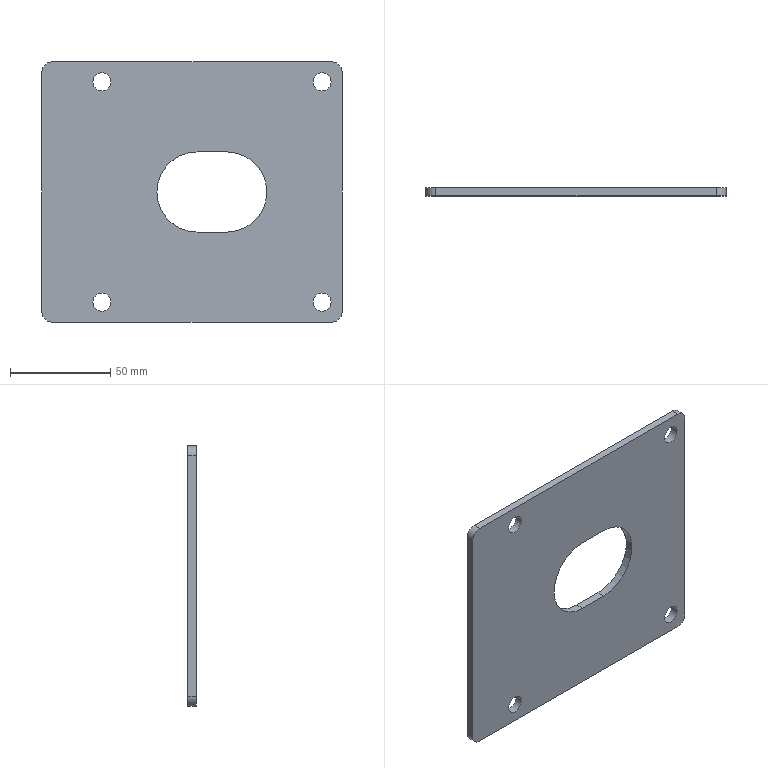Component | SolidWorks | CoverPlate.1_2-1 | 1 solid | 23 faces | box 150 x 4 x 130 mm | volume 69470 mm3 | cylinder 15 | plane 8 | commonest cylinder face diameters 9 x8 10 x4 40 x3
build123d program:
from build123d import *

# Parameters (mm, degrees)
SKETCH1_W           = 130
SKETCH1_H           = 150
BOSS_EXTRUDE1_DEPTH = 4
SKETCH2_R           = 4.5
CUT_EXTRUDE1_DEPTH  = 5
CUT_EXTRUDE2_DEPTH  = 5
FILLET1_R           = 5


with BuildPart() as part:
    # Sketch1 → Boss-Extrude1 (new body)
    with BuildSketch(Plane(origin=(0, 0, 0), x_dir=(1, 0, 0), z_dir=(0, 1, 0))):
        Rectangle(SKETCH1_W, SKETCH1_H)
    extrude(amount=BOSS_EXTRUDE1_DEPTH)

    # Sketch2 → Cut-Extrude1 (cut)
    with BuildSketch(Plane(origin=(0, 4, 0), x_dir=(1, 0, 0), z_dir=(0, 1, 0))):
        with Locations(Location((-55, 65, 0), (0, 0, 270))):
            Circle(SKETCH2_R)
        with Locations(Location((55, 65, 0), (0, 0, 270))):
            Circle(SKETCH2_R)
        with Locations(Location((55, -45, 0), (0, 0, 270))):
            Circle(SKETCH2_R)
        with Locations(Location((-55, -45, 0), (0, 0, 270))):
            Circle(SKETCH2_R)
    extrude(amount=-CUT_EXTRUDE1_DEPTH, mode=Mode.SUBTRACT)

    # Sketch3 → Cut-Extrude2 (cut)
    with BuildSketch(Plane(origin=(0, 4, 0), x_dir=(1, 0, 0), z_dir=(0, 1, 0))):
        with BuildLine():
            Line((-20, 2.5), (-20, 17.5))
            ThreePointArc((-20, 17.5), (0, 37.5), (20, 17.5))
            Line((20, 17.5), (20, 2.5))
            ThreePointArc((20, 2.5), (0, -17.5), (-20, 2.5))
        make_face()
    extrude(amount=-CUT_EXTRUDE2_DEPTH, mode=Mode.SUBTRACT)

    # Fillet1
    fillet1_edges = [part.edges().sort_by_distance(p)[0] for p in [
        (65, 2, 75),
        (-65, 2, 75),
        (-65, 2, -75),
        (65, 2, -75),
    ]]
    fillet(fillet1_edges, radius=FILLET1_R)


solid = part.part

# Placed as in the assembly
solid = solid.moved(Location((-10, 0, -0.4), (0, -90, 0)))
STEP:
#1=CARTESIAN_POINT('',(-1.083,-0.,-0.01575));
#2=VERTEX_POINT('',#1);
#3=CARTESIAN_POINT('',(-0.2953,-0.,0.7717));
#4=VERTEX_POINT('',#3);
#5=CARTESIAN_POINT('',(-0.2953,-0.,-0.01575));
#6=DIRECTION('',(0.,1.,-0.));
#7=DIRECTION('',(-1.,0.,-0.));
#8=AXIS2_PLACEMENT_3D('',#5,#6,#7);
#9=CIRCLE('',#8,0.7874);
#10=EDGE_CURVE('',#2,#4,#9,.T.);
#11=ORIENTED_EDGE('',*,*,#10,.F.);
#12=CARTESIAN_POINT('',(-1.083,0.1575,-0.01575));
#13=VERTEX_POINT('',#12);
#14=CARTESIAN_POINT('',(-1.083,-0.03937,-0.01575));
#15=DIRECTION('',(0.,1.,-0.));
#16=VECTOR('',#15,39.37);
#17=LINE('',#14,#16);
#18=EDGE_CURVE('',#2,#13,#17,.T.);
#19=ORIENTED_EDGE('',*,*,#18,.T.);
#20=CARTESIAN_POINT('',(-0.2953,0.1575,0.7717));
#21=VERTEX_POINT('',#20);
#22=CARTESIAN_POINT('',(-0.2953,0.1575,-0.01575));
#23=DIRECTION('',(0.,1.,-0.));
#24=DIRECTION('',(-1.,0.,-0.));
#25=AXIS2_PLACEMENT_3D('',#22,#23,#24);
#26=CIRCLE('',#25,0.7874);
#27=EDGE_CURVE('',#13,#21,#26,.T.);
#28=ORIENTED_EDGE('',*,*,#27,.T.);
#29=CARTESIAN_POINT('',(-0.2953,-0.03937,0.7717));
#30=DIRECTION('',(0.,1.,-0.));
#31=VECTOR('',#30,39.37);
#32=LINE('',#29,#31);
#33=EDGE_CURVE('',#4,#21,#32,.T.);
#34=ORIENTED_EDGE('',*,*,#33,.F.);
#35=EDGE_LOOP('',(#11,#19,#28,#34));
#36=FACE_OUTER_BOUND('',#35,.T.);
#37=CARTESIAN_POINT('',(-0.2953,-0.03937,-0.01575));
#38=DIRECTION('',(0.,1.,-0.));
#39=DIRECTION('',(-1.,0.,-0.));
#40=AXIS2_PLACEMENT_3D('',#37,#38,#39);
#41=CYLINDRICAL_SURFACE('',#40,0.7874);
#42=ADVANCED_FACE('',(#36),#41,.F.);
#43=CARTESIAN_POINT('',(-1.988,-0.,-2.181));
#44=VERTEX_POINT('',#43);
#45=CARTESIAN_POINT('',(-2.343,-0.,-2.181));
#46=VERTEX_POINT('',#45);
#47=CARTESIAN_POINT('',(-2.165,-0.,-2.181));
#48=DIRECTION('',(0.,1.,-0.));
#49=DIRECTION('',(-1.,0.,0.));
#50=AXIS2_PLACEMENT_3D('',#47,#48,#49);
#51=CIRCLE('',#50,0.1772);
#52=EDGE_CURVE('',#44,#46,#51,.T.);
#53=ORIENTED_EDGE('',*,*,#52,.F.);
#54=CARTESIAN_POINT('',(-1.988,0.1575,-2.181));
#55=VERTEX_POINT('',#54);
#56=CARTESIAN_POINT('',(-1.988,-0.03937,-2.181));
#57=DIRECTION('',(0.,1.,-0.));
#58=VECTOR('',#57,39.37);
#59=LINE('',#56,#58);
#60=EDGE_CURVE('',#44,#55,#59,.T.);
#61=ORIENTED_EDGE('',*,*,#60,.T.);
#62=CARTESIAN_POINT('',(-2.343,0.1575,-2.181));
#63=VERTEX_POINT('',#62);
#64=CARTESIAN_POINT('',(-2.165,0.1575,-2.181));
#65=DIRECTION('',(0.,1.,-0.));
#66=DIRECTION('',(1.,0.,0.));
#67=AXIS2_PLACEMENT_3D('',#64,#65,#66);
#68=CIRCLE('',#67,0.1772);
#69=EDGE_CURVE('',#55,#63,#68,.T.);
#70=ORIENTED_EDGE('',*,*,#69,.T.);
#71=CARTESIAN_POINT('',(-2.343,-0.03937,-2.181));
#72=DIRECTION('',(0.,1.,-0.));
#73=VECTOR('',#72,39.37);
#74=LINE('',#71,#73);
#75=EDGE_CURVE('',#46,#63,#74,.T.);
#76=ORIENTED_EDGE('',*,*,#75,.F.);
#77=EDGE_LOOP('',(#53,#61,#70,#76));
#78=FACE_OUTER_BOUND('',#77,.T.);
#79=CARTESIAN_POINT('',(-2.165,-0.03937,-2.181));
#80=DIRECTION('',(0.,1.,-0.));
#81=DIRECTION('',(-1.,0.,0.));
#82=AXIS2_PLACEMENT_3D('',#79,#80,#81);
#83=CYLINDRICAL_SURFACE('',#82,0.1772);
#84=ADVANCED_FACE('',(#78),#83,.F.);
#85=CARTESIAN_POINT('',(-1.988,-0.,2.15));
#86=VERTEX_POINT('',#85);
#87=CARTESIAN_POINT('',(-2.343,-0.,2.15));
#88=VERTEX_POINT('',#87);
#89=CARTESIAN_POINT('',(-2.165,-0.,2.15));
#90=DIRECTION('',(0.,1.,-0.));
#91=DIRECTION('',(-1.,0.,0.));
#92=AXIS2_PLACEMENT_3D('',#89,#90,#91);
#93=CIRCLE('',#92,0.1772);
#94=EDGE_CURVE('',#86,#88,#93,.T.);
#95=ORIENTED_EDGE('',*,*,#94,.F.);
#96=CARTESIAN_POINT('',(-1.988,0.1575,2.15));
#97=VERTEX_POINT('',#96);
#98=CARTESIAN_POINT('',(-1.988,-0.03937,2.15));
#99=DIRECTION('',(0.,1.,-0.));
#100=VECTOR('',#99,39.37);
#101=LINE('',#98,#100);
#102=EDGE_CURVE('',#86,#97,#101,.T.);
#103=ORIENTED_EDGE('',*,*,#102,.T.);
#104=CARTESIAN_POINT('',(-2.343,0.1575,2.15));
#105=VERTEX_POINT('',#104);
#106=CARTESIAN_POINT('',(-2.165,0.1575,2.15));
#107=DIRECTION('',(0.,1.,-0.));
#108=DIRECTION('',(-1.,0.,0.));
#109=AXIS2_PLACEMENT_3D('',#106,#107,#108);
#110=CIRCLE('',#109,0.1772);
#111=EDGE_CURVE('',#97,#105,#110,.T.);
#112=ORIENTED_EDGE('',*,*,#111,.T.);
#113=CARTESIAN_POINT('',(-2.343,-0.03937,2.15));
#114=DIRECTION('',(0.,1.,-0.));
#115=VECTOR('',#114,39.37);
#116=LINE('',#113,#115);
#117=EDGE_CURVE('',#88,#105,#116,.T.);
#118=ORIENTED_EDGE('',*,*,#117,.F.);
#119=EDGE_LOOP('',(#95,#103,#112,#118));
#120=FACE_OUTER_BOUND('',#119,.T.);
#121=CARTESIAN_POINT('',(-2.165,-0.03937,2.15));
#122=DIRECTION('',(0.,1.,-0.));
#123=DIRECTION('',(-1.,0.,0.));
#124=AXIS2_PLACEMENT_3D('',#121,#122,#123);
#125=CYLINDRICAL_SURFACE('',#124,0.1772);
#126=ADVANCED_FACE('',(#120),#125,.F.);
#127=CARTESIAN_POINT('',(2.343,-0.,2.15));
#128=VERTEX_POINT('',#127);
#129=CARTESIAN_POINT('',(1.988,-0.,2.15));
#130=VERTEX_POINT('',#129);
#131=CARTESIAN_POINT('',(2.165,-0.,2.15));
#132=DIRECTION('',(0.,1.,-0.));
#133=DIRECTION('',(-1.,0.,0.));
#134=AXIS2_PLACEMENT_3D('',#131,#132,#133);
#135=CIRCLE('',#134,0.1772);
#136=EDGE_CURVE('',#128,#130,#135,.T.);
#137=ORIENTED_EDGE('',*,*,#136,.F.);
#138=CARTESIAN_POINT('',(2.343,0.1575,2.15));
#139=VERTEX_POINT('',#138);
#140=CARTESIAN_POINT('',(2.343,-0.03937,2.15));
#141=DIRECTION('',(0.,1.,-0.));
#142=VECTOR('',#141,39.37);
#143=LINE('',#140,#142);
#144=EDGE_CURVE('',#128,#139,#143,.T.);
#145=ORIENTED_EDGE('',*,*,#144,.T.);
#146=CARTESIAN_POINT('',(1.988,0.1575,2.15));
#147=VERTEX_POINT('',#146);
#148=CARTESIAN_POINT('',(2.165,0.1575,2.15));
#149=DIRECTION('',(0.,1.,-0.));
#150=DIRECTION('',(1.,0.,0.));
#151=AXIS2_PLACEMENT_3D('',#148,#149,#150);
#152=CIRCLE('',#151,0.1772);
#153=EDGE_CURVE('',#139,#147,#152,.T.);
#154=ORIENTED_EDGE('',*,*,#153,.T.);
#155=CARTESIAN_POINT('',(1.988,-0.03937,2.15));
#156=DIRECTION('',(0.,1.,-0.));
#157=VECTOR('',#156,39.37);
#158=LINE('',#155,#157);
#159=EDGE_CURVE('',#130,#147,#158,.T.);
#160=ORIENTED_EDGE('',*,*,#159,.F.);
#161=EDGE_LOOP('',(#137,#145,#154,#160));
#162=FACE_OUTER_BOUND('',#161,.T.);
#163=CARTESIAN_POINT('',(2.165,-0.03937,2.15));
#164=DIRECTION('',(0.,1.,-0.));
#165=DIRECTION('',(-1.,0.,0.));
#166=AXIS2_PLACEMENT_3D('',#163,#164,#165);
#167=CYLINDRICAL_SURFACE('',#166,0.1772);
#168=ADVANCED_FACE('',(#162),#167,.F.);
#169=CARTESIAN_POINT('',(2.343,-0.,-2.181));
#170=VERTEX_POINT('',#169);
#171=CARTESIAN_POINT('',(1.988,-0.,-2.181));
#172=VERTEX_POINT('',#171);
#173=CARTESIAN_POINT('',(2.165,-0.,-2.181));
#174=DIRECTION('',(0.,1.,-0.));
#175=DIRECTION('',(-1.,0.,0.));
#176=AXIS2_PLACEMENT_3D('',#173,#174,#175);
#177=CIRCLE('',#176,0.1772);
#178=EDGE_CURVE('',#170,#172,#177,.T.);
#179=ORIENTED_EDGE('',*,*,#178,.F.);
#180=CARTESIAN_POINT('',(2.343,0.1575,-2.181));
#181=VERTEX_POINT('',#180);
#182=CARTESIAN_POINT('',(2.343,-0.03937,-2.181));
#183=DIRECTION('',(0.,1.,-0.));
#184=VECTOR('',#183,39.37);
#185=LINE('',#182,#184);
#186=EDGE_CURVE('',#170,#181,#185,.T.);
#187=ORIENTED_EDGE('',*,*,#186,.T.);
#188=CARTESIAN_POINT('',(1.988,0.1575,-2.181));
#189=VERTEX_POINT('',#188);
#190=CARTESIAN_POINT('',(2.165,0.1575,-2.181));
#191=DIRECTION('',(0.,1.,-0.));
#192=DIRECTION('',(-1.,0.,0.));
#193=AXIS2_PLACEMENT_3D('',#190,#191,#192);
#194=CIRCLE('',#193,0.1772);
#195=EDGE_CURVE('',#181,#189,#194,.T.);
#196=ORIENTED_EDGE('',*,*,#195,.T.);
#197=CARTESIAN_POINT('',(1.988,-0.03937,-2.181));
#198=DIRECTION('',(0.,1.,-0.));
#199=VECTOR('',#198,39.37);
#200=LINE('',#197,#199);
#201=EDGE_CURVE('',#172,#189,#200,.T.);
#202=ORIENTED_EDGE('',*,*,#201,.F.);
#203=EDGE_LOOP('',(#179,#187,#196,#202));
#204=FACE_OUTER_BOUND('',#203,.T.);
#205=CARTESIAN_POINT('',(2.165,-0.03937,-2.181));
#206=DIRECTION('',(0.,1.,-0.));
#207=DIRECTION('',(-1.,0.,0.));
#208=AXIS2_PLACEMENT_3D('',#205,#206,#207);
#209=CYLINDRICAL_SURFACE('',#208,0.1772);
#210=ADVANCED_FACE('',(#204),#209,.F.);
#211=CARTESIAN_POINT('',(-3.15,0.1575,2.543));
#212=VERTEX_POINT('',#211);
#213=CARTESIAN_POINT('',(2.362,0.1575,2.543));
#214=VERTEX_POINT('',#213);
#215=CARTESIAN_POINT('',(2.559,0.1575,2.543));
#216=DIRECTION('',(1.,-0.,0.));
#217=VECTOR('',#216,39.37);
#218=LINE('',#215,#217);
#219=EDGE_CURVE('',#212,#214,#218,.T.);
#220=ORIENTED_EDGE('',*,*,#219,.F.);
#221=CARTESIAN_POINT('',(-3.15,-0.,2.543));
#222=VERTEX_POINT('',#221);
#223=CARTESIAN_POINT('',(-3.15,0.1575,2.543));
#224=DIRECTION('',(-0.,-1.,0.));
#225=VECTOR('',#224,39.37);
#226=LINE('',#223,#225);
#227=EDGE_CURVE('',#212,#222,#226,.T.);
#228=ORIENTED_EDGE('',*,*,#227,.T.);
#229=CARTESIAN_POINT('',(2.362,-0.,2.543));
#230=VERTEX_POINT('',#229);
#231=CARTESIAN_POINT('',(2.559,-0.,2.543));
#232=DIRECTION('',(1.,-0.,0.));
#233=VECTOR('',#232,39.37);
#234=LINE('',#231,#233);
#235=EDGE_CURVE('',#222,#230,#234,.T.);
#236=ORIENTED_EDGE('',*,*,#235,.T.);
#237=CARTESIAN_POINT('',(2.362,0.1575,2.543));
#238=DIRECTION('',(0.,1.,-0.));
#239=VECTOR('',#238,39.37);
#240=LINE('',#237,#239);
#241=EDGE_CURVE('',#230,#214,#240,.T.);
#242=ORIENTED_EDGE('',*,*,#241,.T.);
#243=EDGE_LOOP('',(#220,#228,#236,#242));
#244=FACE_OUTER_BOUND('',#243,.T.);
#245=CARTESIAN_POINT('',(2.559,0.1575,2.543));
#246=DIRECTION('',(0.,-0.,-1.));
#247=DIRECTION('',(-1.,0.,-0.));
#248=AXIS2_PLACEMENT_3D('',#245,#246,#247);
#249=PLANE('',#248);
#250=ADVANCED_FACE('',(#244),#249,.F.);
#251=CARTESIAN_POINT('',(2.559,-0.,2.346));
#252=VERTEX_POINT('',#251);
#253=CARTESIAN_POINT('',(2.559,-0.,-2.378));
#254=VERTEX_POINT('',#253);
#255=CARTESIAN_POINT('',(2.559,-0.,-2.575));
#256=DIRECTION('',(0.,-0.,-1.));
#257=VECTOR('',#256,39.37);
#258=LINE('',#255,#257);
#259=EDGE_CURVE('',#252,#254,#258,.T.);
#260=ORIENTED_EDGE('',*,*,#259,.T.);
#261=CARTESIAN_POINT('',(2.559,0.1575,-2.378));
#262=VERTEX_POINT('',#261);
#263=CARTESIAN_POINT('',(2.559,0.1575,-2.378));
#264=DIRECTION('',(0.,1.,-0.));
#265=VECTOR('',#264,39.37);
#266=LINE('',#263,#265);
#267=EDGE_CURVE('',#254,#262,#266,.T.);
#268=ORIENTED_EDGE('',*,*,#267,.T.);
#269=CARTESIAN_POINT('',(2.559,0.1575,2.346));
#270=VERTEX_POINT('',#269);
#271=CARTESIAN_POINT('',(2.559,0.1575,-2.575));
#272=DIRECTION('',(0.,-0.,-1.));
#273=VECTOR('',#272,39.37);
#274=LINE('',#271,#273);
#275=EDGE_CURVE('',#270,#262,#274,.T.);
#276=ORIENTED_EDGE('',*,*,#275,.F.);
#277=CARTESIAN_POINT('',(2.559,0.1575,2.346));
#278=DIRECTION('',(-0.,-1.,0.));
#279=VECTOR('',#278,39.37);
#280=LINE('',#277,#279);
#281=EDGE_CURVE('',#270,#252,#280,.T.);
#282=ORIENTED_EDGE('',*,*,#281,.T.);
#283=EDGE_LOOP('',(#260,#268,#276,#282));
#284=FACE_OUTER_BOUND('',#283,.T.);
#285=CARTESIAN_POINT('',(2.559,0.1575,-2.575));
#286=DIRECTION('',(-1.,0.,-0.));
#287=DIRECTION('',(-0.,0.,1.));
#288=AXIS2_PLACEMENT_3D('',#285,#286,#287);
#289=PLANE('',#288);
#290=ADVANCED_FACE('',(#284),#289,.F.);
#291=CARTESIAN_POINT('',(2.362,-0.,-2.575));
#292=VERTEX_POINT('',#291);
#293=CARTESIAN_POINT('',(-3.15,-0.,-2.575));
#294=VERTEX_POINT('',#293);
#295=CARTESIAN_POINT('',(2.559,-0.,-2.575));
#296=DIRECTION('',(-1.,0.,-0.));
#297=VECTOR('',#296,39.37);
#298=LINE('',#295,#297);
#299=EDGE_CURVE('',#292,#294,#298,.T.);
#300=ORIENTED_EDGE('',*,*,#299,.T.);
#301=CARTESIAN_POINT('',(-3.15,0.1575,-2.575));
#302=VERTEX_POINT('',#301);
#303=CARTESIAN_POINT('',(-3.15,0.1575,-2.575));
#304=DIRECTION('',(0.,1.,-0.));
#305=VECTOR('',#304,39.37);
#306=LINE('',#303,#305);
#307=EDGE_CURVE('',#294,#302,#306,.T.);
#308=ORIENTED_EDGE('',*,*,#307,.T.);
#309=CARTESIAN_POINT('',(2.362,0.1575,-2.575));
#310=VERTEX_POINT('',#309);
#311=CARTESIAN_POINT('',(2.559,0.1575,-2.575));
#312=DIRECTION('',(-1.,0.,-0.));
#313=VECTOR('',#312,39.37);
#314=LINE('',#311,#313);
#315=EDGE_CURVE('',#310,#302,#314,.T.);
#316=ORIENTED_EDGE('',*,*,#315,.F.);
#317=CARTESIAN_POINT('',(2.362,0.1575,-2.575));
#318=DIRECTION('',(-0.,-1.,0.));
#319=VECTOR('',#318,39.37);
#320=LINE('',#317,#319);
#321=EDGE_CURVE('',#310,#292,#320,.T.);
#322=ORIENTED_EDGE('',*,*,#321,.T.);
#323=EDGE_LOOP('',(#300,#308,#316,#322));
#324=FACE_OUTER_BOUND('',#323,.T.);
#325=CARTESIAN_POINT('',(2.559,0.1575,-2.575));
#326=DIRECTION('',(-0.,0.,1.));
#327=DIRECTION('',(1.,-0.,0.));
#328=AXIS2_PLACEMENT_3D('',#325,#326,#327);
#329=PLANE('',#328);
#330=ADVANCED_FACE('',(#324),#329,.F.);
#331=CARTESIAN_POINT('',(-3.346,0.1575,-2.378));
#332=VERTEX_POINT('',#331);
#333=CARTESIAN_POINT('',(-3.346,0.1575,2.346));
#334=VERTEX_POINT('',#333);
#335=CARTESIAN_POINT('',(-3.346,0.1575,-2.575));
#336=DIRECTION('',(-0.,0.,1.));
#337=VECTOR('',#336,39.37);
#338=LINE('',#335,#337);
#339=EDGE_CURVE('',#332,#334,#338,.T.);
#340=ORIENTED_EDGE('',*,*,#339,.F.);
#341=CARTESIAN_POINT('',(-3.346,-0.,-2.378));
#342=VERTEX_POINT('',#341);
#343=CARTESIAN_POINT('',(-3.346,0.1575,-2.378));
#344=DIRECTION('',(-0.,-1.,0.));
#345=VECTOR('',#344,39.37);
#346=LINE('',#343,#345);
#347=EDGE_CURVE('',#332,#342,#346,.T.);
#348=ORIENTED_EDGE('',*,*,#347,.T.);
#349=CARTESIAN_POINT('',(-3.346,-0.,2.346));
#350=VERTEX_POINT('',#349);
#351=CARTESIAN_POINT('',(-3.346,-0.,-2.575));
#352=DIRECTION('',(-0.,0.,1.));
#353=VECTOR('',#352,39.37);
#354=LINE('',#351,#353);
#355=EDGE_CURVE('',#342,#350,#354,.T.);
#356=ORIENTED_EDGE('',*,*,#355,.T.);
#357=CARTESIAN_POINT('',(-3.346,0.1575,2.346));
#358=DIRECTION('',(0.,1.,-0.));
#359=VECTOR('',#358,39.37);
#360=LINE('',#357,#359);
#361=EDGE_CURVE('',#350,#334,#360,.T.);
#362=ORIENTED_EDGE('',*,*,#361,.T.);
#363=EDGE_LOOP('',(#340,#348,#356,#362));
#364=FACE_OUTER_BOUND('',#363,.T.);
#365=CARTESIAN_POINT('',(-3.346,0.1575,-2.575));
#366=DIRECTION('',(1.,-0.,0.));
#367=DIRECTION('',(0.,-0.,-1.));
#368=AXIS2_PLACEMENT_3D('',#365,#366,#367);
#369=PLANE('',#368);
#370=ADVANCED_FACE('',(#364),#369,.F.);
#371=CARTESIAN_POINT('',(-0.2953,0.1575,-0.8031));
#372=VERTEX_POINT('',#371);
#373=CARTESIAN_POINT('',(-0.2953,0.1575,-0.01575));
#374=DIRECTION('',(0.,1.,-0.));
#375=DIRECTION('',(-1.,0.,-0.));
#376=AXIS2_PLACEMENT_3D('',#373,#374,#375);
#377=CIRCLE('',#376,0.7874);
#378=EDGE_CURVE('',#372,#13,#377,.T.);
#379=ORIENTED_EDGE('',*,*,#378,.F.);
#380=CARTESIAN_POINT('',(0.2953,0.1575,-0.8031));
#381=VERTEX_POINT('',#380);
#382=CARTESIAN_POINT('',(-0.2953,0.1575,-0.8031));
#383=DIRECTION('',(-1.,0.,-0.));
#384=VECTOR('',#383,39.37);
#385=LINE('',#382,#384);
#386=EDGE_CURVE('',#381,#372,#385,.T.);
#387=ORIENTED_EDGE('',*,*,#386,.F.);
#388=CARTESIAN_POINT('',(0.2953,0.1575,0.7717));
#389=VERTEX_POINT('',#388);
#390=CARTESIAN_POINT('',(0.2953,0.1575,-0.01575));
#391=DIRECTION('',(0.,1.,-0.));
#392=DIRECTION('',(-1.,0.,-0.));
#393=AXIS2_PLACEMENT_3D('',#390,#391,#392);
#394=CIRCLE('',#393,0.7874);
#395=EDGE_CURVE('',#389,#381,#394,.T.);
#396=ORIENTED_EDGE('',*,*,#395,.F.);
#397=CARTESIAN_POINT('',(-0.2953,0.1575,0.7717));
#398=DIRECTION('',(1.,-0.,0.));
#399=VECTOR('',#398,39.37);
#400=LINE('',#397,#399);
#401=EDGE_CURVE('',#21,#389,#400,.T.);
#402=ORIENTED_EDGE('',*,*,#401,.F.);
#403=ORIENTED_EDGE('',*,*,#27,.F.);
#404=EDGE_LOOP('',(#379,#387,#396,#402,#403));
#405=FACE_BOUND('',#404,.T.);
#406=CARTESIAN_POINT('',(-2.165,0.1575,-2.181));
#407=DIRECTION('',(0.,1.,-0.));
#408=DIRECTION('',(1.,0.,0.));
#409=AXIS2_PLACEMENT_3D('',#406,#407,#408);
#410=CIRCLE('',#409,0.1772);
#411=EDGE_CURVE('',#63,#55,#410,.T.);
#412=ORIENTED_EDGE('',*,*,#411,.F.);
#413=ORIENTED_EDGE('',*,*,#69,.F.);
#414=EDGE_LOOP('',(#412,#413));
#415=FACE_BOUND('',#414,.T.);
#416=CARTESIAN_POINT('',(-2.165,0.1575,2.15));
#417=DIRECTION('',(0.,1.,-0.));
#418=DIRECTION('',(-1.,0.,0.));
#419=AXIS2_PLACEMENT_3D('',#416,#417,#418);
#420=CIRCLE('',#419,0.1772);
#421=EDGE_CURVE('',#105,#97,#420,.T.);
#422=ORIENTED_EDGE('',*,*,#421,.F.);
#423=ORIENTED_EDGE('',*,*,#111,.F.);
#424=EDGE_LOOP('',(#422,#423));
#425=FACE_BOUND('',#424,.T.);
#426=CARTESIAN_POINT('',(2.165,0.1575,2.15));
#427=DIRECTION('',(0.,1.,-0.));
#428=DIRECTION('',(1.,0.,0.));
#429=AXIS2_PLACEMENT_3D('',#426,#427,#428);
#430=CIRCLE('',#429,0.1772);
#431=EDGE_CURVE('',#147,#139,#430,.T.);
#432=ORIENTED_EDGE('',*,*,#431,.F.);
#433=ORIENTED_EDGE('',*,*,#153,.F.);
#434=EDGE_LOOP('',(#432,#433));
#435=FACE_BOUND('',#434,.T.);
#436=CARTESIAN_POINT('',(2.165,0.1575,-2.181));
#437=DIRECTION('',(0.,1.,-0.));
#438=DIRECTION('',(-1.,0.,0.));
#439=AXIS2_PLACEMENT_3D('',#436,#437,#438);
#440=CIRCLE('',#439,0.1772);
#441=EDGE_CURVE('',#189,#181,#440,.T.);
#442=ORIENTED_EDGE('',*,*,#441,.F.);
#443=ORIENTED_EDGE('',*,*,#195,.F.);
#444=EDGE_LOOP('',(#442,#443));
#445=FACE_BOUND('',#444,.T.);
#446=ORIENTED_EDGE('',*,*,#315,.T.);
#447=CARTESIAN_POINT('',(-3.15,0.1575,-2.378));
#448=DIRECTION('',(0.,1.,-0.));
#449=DIRECTION('',(-1.,0.,0.));
#450=AXIS2_PLACEMENT_3D('',#447,#448,#449);
#451=CIRCLE('',#450,0.1969);
#452=EDGE_CURVE('',#302,#332,#451,.T.);
#453=ORIENTED_EDGE('',*,*,#452,.T.);
#454=ORIENTED_EDGE('',*,*,#339,.T.);
#455=CARTESIAN_POINT('',(-3.15,0.1575,2.346));
#456=DIRECTION('',(0.,1.,-0.));
#457=DIRECTION('',(-1.,0.,0.));
#458=AXIS2_PLACEMENT_3D('',#455,#456,#457);
#459=CIRCLE('',#458,0.1969);
#460=EDGE_CURVE('',#334,#212,#459,.T.);
#461=ORIENTED_EDGE('',*,*,#460,.T.);
#462=ORIENTED_EDGE('',*,*,#219,.T.);
#463=CARTESIAN_POINT('',(2.362,0.1575,2.346));
#464=DIRECTION('',(0.,1.,-0.));
#465=DIRECTION('',(-1.,0.,0.));
#466=AXIS2_PLACEMENT_3D('',#463,#464,#465);
#467=CIRCLE('',#466,0.1969);
#468=EDGE_CURVE('',#214,#270,#467,.T.);
#469=ORIENTED_EDGE('',*,*,#468,.T.);
#470=ORIENTED_EDGE('',*,*,#275,.T.);
#471=CARTESIAN_POINT('',(2.362,0.1575,-2.378));
#472=DIRECTION('',(0.,1.,-0.));
#473=DIRECTION('',(-1.,0.,0.));
#474=AXIS2_PLACEMENT_3D('',#471,#472,#473);
#475=CIRCLE('',#474,0.1969);
#476=EDGE_CURVE('',#262,#310,#475,.T.);
#477=ORIENTED_EDGE('',*,*,#476,.T.);
#478=EDGE_LOOP('',(#446,#453,#454,#461,#462,#469,#470,#477));
#479=FACE_OUTER_BOUND('',#478,.T.);
#480=CARTESIAN_POINT('',(-0.3937,0.1575,-0.01575));
#481=DIRECTION('',(0.,1.,-0.));
#482=DIRECTION('',(-1.,0.,-0.));
#483=AXIS2_PLACEMENT_3D('',#480,#481,#482);
#484=PLANE('',#483);
#485=ADVANCED_FACE('',(#405,#415,#425,#435,#445,#479),#484,.T.);
#486=CARTESIAN_POINT('',(0.2953,-0.,-0.8031));
#487=VERTEX_POINT('',#486);
#488=CARTESIAN_POINT('',(-0.2953,-0.,-0.8031));
#489=VERTEX_POINT('',#488);
#490=CARTESIAN_POINT('',(-0.3937,-0.,-0.8031));
#491=DIRECTION('',(-1.,0.,-0.));
#492=VECTOR('',#491,39.37);
#493=LINE('',#490,#492);
#494=EDGE_CURVE('',#487,#489,#493,.T.);
#495=ORIENTED_EDGE('',*,*,#494,.T.);
#496=CARTESIAN_POINT('',(-0.2953,-0.,-0.01575));
#497=DIRECTION('',(0.,1.,-0.));
#498=DIRECTION('',(-1.,0.,-0.));
#499=AXIS2_PLACEMENT_3D('',#496,#497,#498);
#500=CIRCLE('',#499,0.7874);
#501=EDGE_CURVE('',#489,#2,#500,.T.);
#502=ORIENTED_EDGE('',*,*,#501,.T.);
#503=ORIENTED_EDGE('',*,*,#10,.T.);
#504=CARTESIAN_POINT('',(0.2953,-0.,0.7717));
#505=VERTEX_POINT('',#504);
#506=CARTESIAN_POINT('',(-0.3937,-0.,0.7717));
#507=DIRECTION('',(1.,-0.,0.));
#508=VECTOR('',#507,39.37);
#509=LINE('',#506,#508);
#510=EDGE_CURVE('',#4,#505,#509,.T.);
#511=ORIENTED_EDGE('',*,*,#510,.T.);
#512=CARTESIAN_POINT('',(0.2953,-0.,-0.01575));
#513=DIRECTION('',(0.,1.,-0.));
#514=DIRECTION('',(-1.,0.,-0.));
#515=AXIS2_PLACEMENT_3D('',#512,#513,#514);
#516=CIRCLE('',#515,0.7874);
#517=EDGE_CURVE('',#505,#487,#516,.T.);
#518=ORIENTED_EDGE('',*,*,#517,.T.);
#519=EDGE_LOOP('',(#495,#502,#503,#511,#518));
#520=FACE_BOUND('',#519,.T.);
#521=CARTESIAN_POINT('',(-2.165,-0.,-2.181));
#522=DIRECTION('',(0.,1.,-0.));
#523=DIRECTION('',(-1.,0.,0.));
#524=AXIS2_PLACEMENT_3D('',#521,#522,#523);
#525=CIRCLE('',#524,0.1772);
#526=EDGE_CURVE('',#46,#44,#525,.T.);
#527=ORIENTED_EDGE('',*,*,#526,.T.);
#528=ORIENTED_EDGE('',*,*,#52,.T.);
#529=EDGE_LOOP('',(#527,#528));
#530=FACE_BOUND('',#529,.T.);
#531=CARTESIAN_POINT('',(-2.165,-0.,2.15));
#532=DIRECTION('',(0.,1.,-0.));
#533=DIRECTION('',(-1.,0.,0.));
#534=AXIS2_PLACEMENT_3D('',#531,#532,#533);
#535=CIRCLE('',#534,0.1772);
#536=EDGE_CURVE('',#88,#86,#535,.T.);
#537=ORIENTED_EDGE('',*,*,#536,.T.);
#538=ORIENTED_EDGE('',*,*,#94,.T.);
#539=EDGE_LOOP('',(#537,#538));
#540=FACE_BOUND('',#539,.T.);
#541=CARTESIAN_POINT('',(2.165,-0.,2.15));
#542=DIRECTION('',(0.,1.,-0.));
#543=DIRECTION('',(-1.,0.,0.));
#544=AXIS2_PLACEMENT_3D('',#541,#542,#543);
#545=CIRCLE('',#544,0.1772);
#546=EDGE_CURVE('',#130,#128,#545,.T.);
#547=ORIENTED_EDGE('',*,*,#546,.T.);
#548=ORIENTED_EDGE('',*,*,#136,.T.);
#549=EDGE_LOOP('',(#547,#548));
#550=FACE_BOUND('',#549,.T.);
#551=CARTESIAN_POINT('',(2.165,-0.,-2.181));
#552=DIRECTION('',(0.,1.,-0.));
#553=DIRECTION('',(-1.,0.,0.));
#554=AXIS2_PLACEMENT_3D('',#551,#552,#553);
#555=CIRCLE('',#554,0.1772);
#556=EDGE_CURVE('',#172,#170,#555,.T.);
#557=ORIENTED_EDGE('',*,*,#556,.T.);
#558=ORIENTED_EDGE('',*,*,#178,.T.);
#559=EDGE_LOOP('',(#557,#558));
#560=FACE_BOUND('',#559,.T.);
#561=ORIENTED_EDGE('',*,*,#355,.F.);
#562=CARTESIAN_POINT('',(-3.15,-0.,-2.378));
#563=DIRECTION('',(-0.,-1.,0.));
#564=DIRECTION('',(-1.,0.,0.));
#565=AXIS2_PLACEMENT_3D('',#562,#563,#564);
#566=CIRCLE('',#565,0.1969);
#567=EDGE_CURVE('',#342,#294,#566,.T.);
#568=ORIENTED_EDGE('',*,*,#567,.T.);
#569=ORIENTED_EDGE('',*,*,#299,.F.);
#570=CARTESIAN_POINT('',(2.362,-0.,-2.378));
#571=DIRECTION('',(-0.,-1.,0.));
#572=DIRECTION('',(-1.,0.,0.));
#573=AXIS2_PLACEMENT_3D('',#570,#571,#572);
#574=CIRCLE('',#573,0.1969);
#575=EDGE_CURVE('',#292,#254,#574,.T.);
#576=ORIENTED_EDGE('',*,*,#575,.T.);
#577=ORIENTED_EDGE('',*,*,#259,.F.);
#578=CARTESIAN_POINT('',(2.362,-0.,2.346));
#579=DIRECTION('',(-0.,-1.,0.));
#580=DIRECTION('',(-1.,0.,0.));
#581=AXIS2_PLACEMENT_3D('',#578,#579,#580);
#582=CIRCLE('',#581,0.1969);
#583=EDGE_CURVE('',#252,#230,#582,.T.);
#584=ORIENTED_EDGE('',*,*,#583,.T.);
#585=ORIENTED_EDGE('',*,*,#235,.F.);
#586=CARTESIAN_POINT('',(-3.15,-0.,2.346));
#587=DIRECTION('',(-0.,-1.,0.));
#588=DIRECTION('',(-1.,0.,0.));
#589=AXIS2_PLACEMENT_3D('',#586,#587,#588);
#590=CIRCLE('',#589,0.1969);
#591=EDGE_CURVE('',#222,#350,#590,.T.);
#592=ORIENTED_EDGE('',*,*,#591,.T.);
#593=EDGE_LOOP('',(#561,#568,#569,#576,#577,#584,#585,#592));
#594=FACE_OUTER_BOUND('',#593,.T.);
#595=CARTESIAN_POINT('',(-0.3937,-0.,-0.01575));
#596=DIRECTION('',(0.,1.,-0.));
#597=DIRECTION('',(-1.,0.,-0.));
#598=AXIS2_PLACEMENT_3D('',#595,#596,#597);
#599=PLANE('',#598);
#600=ADVANCED_FACE('',(#520,#530,#540,#550,#560,#594),#599,.F.);
#601=ORIENTED_EDGE('',*,*,#186,.F.);
#602=ORIENTED_EDGE('',*,*,#556,.F.);
#603=ORIENTED_EDGE('',*,*,#201,.T.);
#604=ORIENTED_EDGE('',*,*,#441,.T.);
#605=EDGE_LOOP('',(#601,#602,#603,#604));
#606=FACE_OUTER_BOUND('',#605,.T.);
#607=CARTESIAN_POINT('',(2.165,-0.03937,-2.181));
#608=DIRECTION('',(0.,1.,-0.));
#609=DIRECTION('',(-1.,0.,0.));
#610=AXIS2_PLACEMENT_3D('',#607,#608,#609);
#611=CYLINDRICAL_SURFACE('',#610,0.1772);
#612=ADVANCED_FACE('',(#606),#611,.F.);
#613=ORIENTED_EDGE('',*,*,#144,.F.);
#614=ORIENTED_EDGE('',*,*,#546,.F.);
#615=ORIENTED_EDGE('',*,*,#159,.T.);
#616=ORIENTED_EDGE('',*,*,#431,.T.);
#617=EDGE_LOOP('',(#613,#614,#615,#616));
#618=FACE_OUTER_BOUND('',#617,.T.);
#619=CARTESIAN_POINT('',(2.165,-0.03937,2.15));
#620=DIRECTION('',(0.,1.,-0.));
#621=DIRECTION('',(-1.,0.,0.));
#622=AXIS2_PLACEMENT_3D('',#619,#620,#621);
#623=CYLINDRICAL_SURFACE('',#622,0.1772);
#624=ADVANCED_FACE('',(#618),#623,.F.);
#625=ORIENTED_EDGE('',*,*,#102,.F.);
#626=ORIENTED_EDGE('',*,*,#536,.F.);
#627=ORIENTED_EDGE('',*,*,#117,.T.);
#628=ORIENTED_EDGE('',*,*,#421,.T.);
#629=EDGE_LOOP('',(#625,#626,#627,#628));
#630=FACE_OUTER_BOUND('',#629,.T.);
#631=CARTESIAN_POINT('',(-2.165,-0.03937,2.15));
#632=DIRECTION('',(0.,1.,-0.));
#633=DIRECTION('',(-1.,0.,0.));
#634=AXIS2_PLACEMENT_3D('',#631,#632,#633);
#635=CYLINDRICAL_SURFACE('',#634,0.1772);
#636=ADVANCED_FACE('',(#630),#635,.F.);
#637=ORIENTED_EDGE('',*,*,#60,.F.);
#638=ORIENTED_EDGE('',*,*,#526,.F.);
#639=ORIENTED_EDGE('',*,*,#75,.T.);
#640=ORIENTED_EDGE('',*,*,#411,.T.);
#641=EDGE_LOOP('',(#637,#638,#639,#640));
#642=FACE_OUTER_BOUND('',#641,.T.);
#643=CARTESIAN_POINT('',(-2.165,-0.03937,-2.181));
#644=DIRECTION('',(0.,1.,-0.));
#645=DIRECTION('',(-1.,0.,0.));
#646=AXIS2_PLACEMENT_3D('',#643,#644,#645);
#647=CYLINDRICAL_SURFACE('',#646,0.1772);
#648=ADVANCED_FACE('',(#642),#647,.F.);
#649=ORIENTED_EDGE('',*,*,#18,.F.);
#650=ORIENTED_EDGE('',*,*,#501,.F.);
#651=CARTESIAN_POINT('',(-0.2953,-0.03937,-0.8031));
#652=DIRECTION('',(0.,1.,-0.));
#653=VECTOR('',#652,39.37);
#654=LINE('',#651,#653);
#655=EDGE_CURVE('',#489,#372,#654,.T.);
#656=ORIENTED_EDGE('',*,*,#655,.T.);
#657=ORIENTED_EDGE('',*,*,#378,.T.);
#658=EDGE_LOOP('',(#649,#650,#656,#657));
#659=FACE_OUTER_BOUND('',#658,.T.);
#660=CARTESIAN_POINT('',(-0.2953,-0.03937,-0.01575));
#661=DIRECTION('',(0.,1.,-0.));
#662=DIRECTION('',(-1.,0.,-0.));
#663=AXIS2_PLACEMENT_3D('',#660,#661,#662);
#664=CYLINDRICAL_SURFACE('',#663,0.7874);
#665=ADVANCED_FACE('',(#659),#664,.F.);
#666=CARTESIAN_POINT('',(0.2953,-0.03937,-0.8031));
#667=DIRECTION('',(0.,1.,-0.));
#668=VECTOR('',#667,39.37);
#669=LINE('',#666,#668);
#670=EDGE_CURVE('',#487,#381,#669,.T.);
#671=ORIENTED_EDGE('',*,*,#670,.T.);
#672=ORIENTED_EDGE('',*,*,#386,.T.);
#673=ORIENTED_EDGE('',*,*,#655,.F.);
#674=ORIENTED_EDGE('',*,*,#494,.F.);
#675=EDGE_LOOP('',(#671,#672,#673,#674));
#676=FACE_OUTER_BOUND('',#675,.T.);
#677=CARTESIAN_POINT('',(-0.2953,-0.03937,-0.8031));
#678=DIRECTION('',(0.,-0.,-1.));
#679=DIRECTION('',(-1.,0.,-0.));
#680=AXIS2_PLACEMENT_3D('',#677,#678,#679);
#681=PLANE('',#680);
#682=ADVANCED_FACE('',(#676),#681,.F.);
#683=CARTESIAN_POINT('',(0.2953,-0.03937,0.7717));
#684=DIRECTION('',(0.,1.,-0.));
#685=VECTOR('',#684,39.37);
#686=LINE('',#683,#685);
#687=EDGE_CURVE('',#505,#389,#686,.T.);
#688=ORIENTED_EDGE('',*,*,#687,.T.);
#689=ORIENTED_EDGE('',*,*,#395,.T.);
#690=ORIENTED_EDGE('',*,*,#670,.F.);
#691=ORIENTED_EDGE('',*,*,#517,.F.);
#692=EDGE_LOOP('',(#688,#689,#690,#691));
#693=FACE_OUTER_BOUND('',#692,.T.);
#694=CARTESIAN_POINT('',(0.2953,-0.03937,-0.01575));
#695=DIRECTION('',(0.,1.,-0.));
#696=DIRECTION('',(-1.,0.,-0.));
#697=AXIS2_PLACEMENT_3D('',#694,#695,#696);
#698=CYLINDRICAL_SURFACE('',#697,0.7874);
#699=ADVANCED_FACE('',(#693),#698,.F.);
#700=ORIENTED_EDGE('',*,*,#33,.T.);
#701=ORIENTED_EDGE('',*,*,#401,.T.);
#702=ORIENTED_EDGE('',*,*,#687,.F.);
#703=ORIENTED_EDGE('',*,*,#510,.F.);
#704=EDGE_LOOP('',(#700,#701,#702,#703));
#705=FACE_OUTER_BOUND('',#704,.T.);
#706=CARTESIAN_POINT('',(-0.2953,-0.03937,0.7717));
#707=DIRECTION('',(-0.,0.,1.));
#708=DIRECTION('',(1.,-0.,0.));
#709=AXIS2_PLACEMENT_3D('',#706,#707,#708);
#710=PLANE('',#709);
#711=ADVANCED_FACE('',(#705),#710,.F.);
#712=ORIENTED_EDGE('',*,*,#452,.F.);
#713=ORIENTED_EDGE('',*,*,#307,.F.);
#714=ORIENTED_EDGE('',*,*,#567,.F.);
#715=ORIENTED_EDGE('',*,*,#347,.F.);
#716=EDGE_LOOP('',(#712,#713,#714,#715));
#717=FACE_OUTER_BOUND('',#716,.T.);
#718=CARTESIAN_POINT('',(-3.15,0.1575,-2.378));
#719=DIRECTION('',(-0.,-1.,0.));
#720=DIRECTION('',(1.,0.,0.));
#721=AXIS2_PLACEMENT_3D('',#718,#719,#720);
#722=CYLINDRICAL_SURFACE('',#721,0.1969);
#723=ADVANCED_FACE('',(#717),#722,.T.);
#724=ORIENTED_EDGE('',*,*,#460,.F.);
#725=ORIENTED_EDGE('',*,*,#361,.F.);
#726=ORIENTED_EDGE('',*,*,#591,.F.);
#727=ORIENTED_EDGE('',*,*,#227,.F.);
#728=EDGE_LOOP('',(#724,#725,#726,#727));
#729=FACE_OUTER_BOUND('',#728,.T.);
#730=CARTESIAN_POINT('',(-3.15,0.1575,2.346));
#731=DIRECTION('',(-0.,-1.,0.));
#732=DIRECTION('',(1.,0.,0.));
#733=AXIS2_PLACEMENT_3D('',#730,#731,#732);
#734=CYLINDRICAL_SURFACE('',#733,0.1969);
#735=ADVANCED_FACE('',(#729),#734,.T.);
#736=ORIENTED_EDGE('',*,*,#476,.F.);
#737=ORIENTED_EDGE('',*,*,#267,.F.);
#738=ORIENTED_EDGE('',*,*,#575,.F.);
#739=ORIENTED_EDGE('',*,*,#321,.F.);
#740=EDGE_LOOP('',(#736,#737,#738,#739));
#741=FACE_OUTER_BOUND('',#740,.T.);
#742=CARTESIAN_POINT('',(2.362,0.1575,-2.378));
#743=DIRECTION('',(-0.,-1.,0.));
#744=DIRECTION('',(1.,0.,0.));
#745=AXIS2_PLACEMENT_3D('',#742,#743,#744);
#746=CYLINDRICAL_SURFACE('',#745,0.1969);
#747=ADVANCED_FACE('',(#741),#746,.T.);
#748=ORIENTED_EDGE('',*,*,#468,.F.);
#749=ORIENTED_EDGE('',*,*,#241,.F.);
#750=ORIENTED_EDGE('',*,*,#583,.F.);
#751=ORIENTED_EDGE('',*,*,#281,.F.);
#752=EDGE_LOOP('',(#748,#749,#750,#751));
#753=FACE_OUTER_BOUND('',#752,.T.);
#754=CARTESIAN_POINT('',(2.362,0.1575,2.346));
#755=DIRECTION('',(-0.,-1.,0.));
#756=DIRECTION('',(1.,0.,0.));
#757=AXIS2_PLACEMENT_3D('',#754,#755,#756);
#758=CYLINDRICAL_SURFACE('',#757,0.1969);
#759=ADVANCED_FACE('',(#753),#758,.T.);
#760=CLOSED_SHELL('',(#42,#84,#126,#168,#210,#250,#290,#330,#370,#485,#600,#612,#624,#636,#648,#665,#682,#699,#711,#723,#735,#747,#759));
#761=MANIFOLD_SOLID_BREP('',#760);
#762=CARTESIAN_POINT('',(0.,0.,0.));
#763=DIRECTION('',(0.,0.,1.));
#764=DIRECTION('',(1.,0.,0.));
#765=AXIS2_PLACEMENT_3D('',#762,#763,#764);
#766=(LENGTH_UNIT()NAMED_UNIT(*)SI_UNIT($,.METRE.));
#767=LENGTH_MEASURE_WITH_UNIT(LENGTH_MEASURE(0.0254),#766);
#768=DIMENSIONAL_EXPONENTS(1.,0.,0.,0.,0.,0.,0.);
#769=(CONVERSION_BASED_UNIT('',#767)LENGTH_UNIT()NAMED_UNIT(#768));
#770=UNCERTAINTY_MEASURE_WITH_UNIT(LENGTH_MEASURE(0.00001),#769,'','');
#771=(NAMED_UNIT(*)PLANE_ANGLE_UNIT()SI_UNIT($,.RADIAN.));
#772=(NAMED_UNIT(*)SI_UNIT($,.STERADIAN.)SOLID_ANGLE_UNIT());
#773=(GEOMETRIC_REPRESENTATION_CONTEXT(3)GLOBAL_UNCERTAINTY_ASSIGNED_CONTEXT((#770))GLOBAL_UNIT_ASSIGNED_CONTEXT((#769,#771,#772))REPRESENTATION_CONTEXT('',''));
#774=ADVANCED_BREP_SHAPE_REPRESENTATION('',(#761,#765),#773);
#775=COLOUR_RGB('',0.7922,0.8196,0.9333);
#776=FILL_AREA_STYLE_COLOUR('',#775);
#777=FILL_AREA_STYLE('',(#776));
#778=SURFACE_STYLE_FILL_AREA(#777);
#779=SURFACE_SIDE_STYLE('',(#778));
#780=SURFACE_STYLE_USAGE(.BOTH.,#779);
#781=PRESENTATION_STYLE_ASSIGNMENT((#780));
#782=STYLED_ITEM('',(#781),#761);
#783=(LENGTH_UNIT()NAMED_UNIT(*)SI_UNIT($,.METRE.));
#784=LENGTH_MEASURE_WITH_UNIT(LENGTH_MEASURE(0.0254),#783);
#785=DIMENSIONAL_EXPONENTS(1.,0.,0.,0.,0.,0.,0.);
#786=(CONVERSION_BASED_UNIT('',#784)LENGTH_UNIT()NAMED_UNIT(#785));
#787=UNCERTAINTY_MEASURE_WITH_UNIT(LENGTH_MEASURE(0.00001),#786,'','');
#788=(NAMED_UNIT(*)PLANE_ANGLE_UNIT()SI_UNIT($,.RADIAN.));
#789=(NAMED_UNIT(*)SI_UNIT($,.STERADIAN.)SOLID_ANGLE_UNIT());
#790=(GEOMETRIC_REPRESENTATION_CONTEXT(3)GLOBAL_UNCERTAINTY_ASSIGNED_CONTEXT((#787))GLOBAL_UNIT_ASSIGNED_CONTEXT((#786,#788,#789))REPRESENTATION_CONTEXT('',''));
#791=MECHANICAL_DESIGN_GEOMETRIC_PRESENTATION_REPRESENTATION('',(#782),#790);
#792=PRESENTATION_LAYER_ASSIGNMENT('','',(#782));